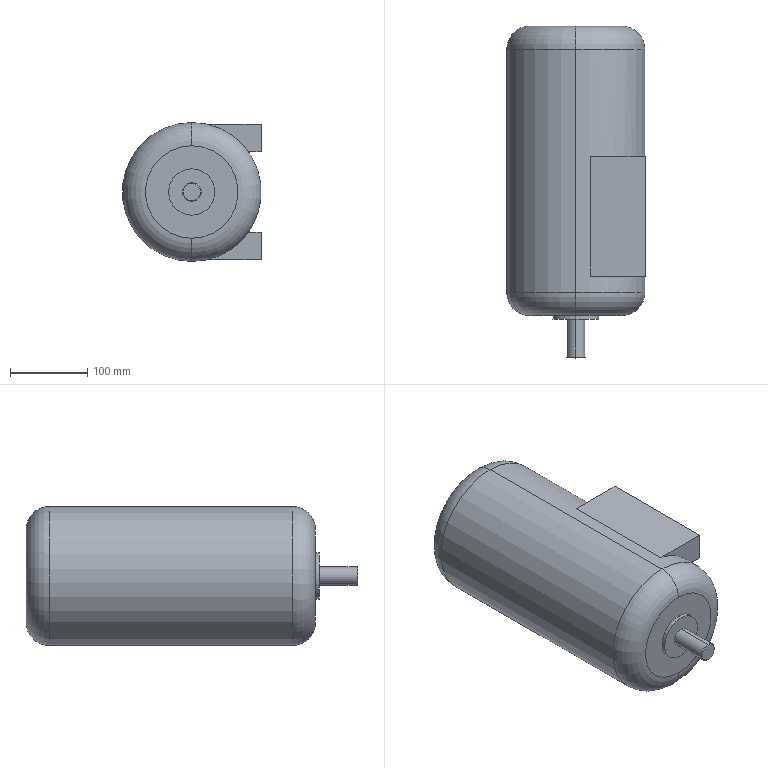Component | SolidWorks | YBBP-903-2-1.5Motor-1 | 1 solid | 26 faces | box 180 x 430 x 180 mm | volume 9782675 mm3 | plane 14 | cylinder 6 | torus 4 | cone 2 | commonest cylinder face diameters 60 x2 24 x2 180 x2 | material 45
build123d program:
from build123d import *

# Parameters (mm, degrees)
BOSS_EXTRUDE1_REACH      = 476.763
BOSS_EXTRUDE1_END_RADIUS = 90
SKETCH2_W                = 155
SKETCH2_H                = 36
FILLET1_R                = 30
CHAMFER1_SIZE            = 1


with BuildPart() as part:
    # Sketch1 → Revolve1 (revolve)
    with BuildSketch(Plane.XY, mode=Mode.PRIVATE) as revolve1_sk:
        Polygon((0, 0), (0, 12), (50, 12), (50, 30), (55, 30), (55, 90), (430, 90), (430, 0), align=None)
    revolve(revolve1_sk.sketch.rotate(Axis((0, 0, 0), (1, 0, 0)), 90), axis=Axis((0, 0, 0), (1, 0, 0)))

    # Boss-Extrude1: up to this cylinder (the profile starts outside it)
    boss_extrude1_end = Plane(origin=(183.5, 0, 0), z_dir=(-1, 0, 0)) * Cylinder(BOSS_EXTRUDE1_END_RADIUS, 1134.526, mode=Mode.PRIVATE)
    # Sketch2 → Boss-Extrude1 (add, up to the surface)
    with BuildSketch(Plane(origin=(0, -90, 0), x_dir=(1, 0, 0), z_dir=(0, 1, 0)), mode=Mode.PRIVATE) as boss_extrude1_sk1:
        with Locations((183.5, -70)):
            Rectangle(SKETCH2_W, SKETCH2_H)
    boss_extrude1_tool1 = extrude(boss_extrude1_sk1.sketch, amount=BOSS_EXTRUDE1_REACH, mode=Mode.PRIVATE) - boss_extrude1_end
    add(boss_extrude1_tool1.solids().sort_by_distance((183.5, -90, 70))[0])
    # Sketch2 → Boss-Extrude1 (add, up to the surface)
    with BuildSketch(Plane(origin=(0, -90, 0), x_dir=(1, 0, 0), z_dir=(0, 1, 0)), mode=Mode.PRIVATE) as boss_extrude1_sk2:
        with Locations((183.5, 70)):
            Rectangle(SKETCH2_W, SKETCH2_H)
    boss_extrude1_tool2 = extrude(boss_extrude1_sk2.sketch, amount=BOSS_EXTRUDE1_REACH, mode=Mode.PRIVATE) - boss_extrude1_end
    add(boss_extrude1_tool2.solids().sort_by_distance((183.5, -90, -70))[0])

    # Fillet1
    fillet1_edges = [part.edges().sort_by_distance(p)[0] for p in [
        (430, 0, -90),
        (55, 0, -90),
    ]]
    fillet(fillet1_edges, radius=FILLET1_R)

    # Chamfer1
    chamfer1_edges = [part.edges().sort_by_distance(p)[0] for p in [
        (0, 0, -12),
    ]]
    chamfer(chamfer1_edges, length=CHAMFER1_SIZE)


solid = part.part

# Placed as in the assembly
solid = solid.moved(Location((-371.359, -392.185, 1412), (0, 0, 90)))
STEP:
#1=COLOUR_RGB('',0.7922,0.8196,0.9333);
#2=FILL_AREA_STYLE_COLOUR('',#1);
#3=FILL_AREA_STYLE('',(#2));
#4=SURFACE_STYLE_FILL_AREA(#3);
#5=SURFACE_SIDE_STYLE('',(#4));
#6=SURFACE_STYLE_USAGE(.BOTH.,#5);
#7=PRESENTATION_STYLE_ASSIGNMENT((#6));
#8=CARTESIAN_POINT('',(-14.62,-15.44,56.024));
#9=VERTEX_POINT('',#8);
#10=CARTESIAN_POINT('',(-14.62,-15.44,55.157));
#11=VERTEX_POINT('',#10);
#12=CARTESIAN_POINT('',(-14.62,-15.44,55.591));
#13=DIRECTION('',(-0.,-1.,0.));
#14=DIRECTION('',(0.,0.,-1.));
#15=AXIS2_PLACEMENT_3D('',#12,#13,#14);
#16=CIRCLE('',#15,0.4331);
#17=EDGE_CURVE('',#9,#11,#16,.T.);
#18=ORIENTED_EDGE('',*,*,#17,.F.);
#19=CARTESIAN_POINT('',(-14.62,-15.401,56.063));
#20=VERTEX_POINT('',#19);
#21=CARTESIAN_POINT('',(-14.62,-15.44,56.024));
#22=DIRECTION('',(-0.,0.7071,0.7071));
#23=VECTOR('',#22,39.37);
#24=LINE('',#21,#23);
#25=EDGE_CURVE('',#9,#20,#24,.T.);
#26=ORIENTED_EDGE('',*,*,#25,.T.);
#27=CARTESIAN_POINT('',(-14.62,-15.401,55.118));
#28=VERTEX_POINT('',#27);
#29=CARTESIAN_POINT('',(-14.62,-15.401,55.591));
#30=DIRECTION('',(0.,1.,0.));
#31=DIRECTION('',(0.,0.,-1.));
#32=AXIS2_PLACEMENT_3D('',#29,#30,#31);
#33=CIRCLE('',#32,0.4724);
#34=EDGE_CURVE('',#28,#20,#33,.T.);
#35=ORIENTED_EDGE('',*,*,#34,.F.);
#36=CARTESIAN_POINT('',(-14.62,-15.44,55.157));
#37=DIRECTION('',(0.,0.7071,-0.7071));
#38=VECTOR('',#37,39.37);
#39=LINE('',#36,#38);
#40=EDGE_CURVE('',#11,#28,#39,.T.);
#41=ORIENTED_EDGE('',*,*,#40,.F.);
#42=EDGE_LOOP('',(#18,#26,#35,#41));
#43=FACE_OUTER_BOUND('',#42,.T.);
#44=CARTESIAN_POINT('',(-14.62,-15.44,55.591));
#45=DIRECTION('',(0.,1.,0.));
#46=DIRECTION('',(0.,0.,-1.));
#47=AXIS2_PLACEMENT_3D('',#44,#45,#46);
#48=CONICAL_SURFACE('',#47,0.4331,0.7854);
#49=ADVANCED_FACE('',(#43),#48,.T.);
#50=CARTESIAN_POINT('',(-14.62,1.489,53.228));
#51=VERTEX_POINT('',#50);
#52=CARTESIAN_POINT('',(-14.62,1.489,57.953));
#53=VERTEX_POINT('',#52);
#54=CARTESIAN_POINT('',(-14.62,1.489,55.591));
#55=DIRECTION('',(0.,1.,0.));
#56=DIRECTION('',(0.,0.,1.));
#57=AXIS2_PLACEMENT_3D('',#54,#55,#56);
#58=CIRCLE('',#57,2.362);
#59=EDGE_CURVE('',#51,#53,#58,.T.);
#60=ORIENTED_EDGE('',*,*,#59,.F.);
#61=CARTESIAN_POINT('',(-14.62,0.3077,52.047));
#62=VERTEX_POINT('',#61);
#63=CARTESIAN_POINT('',(-14.62,0.3077,53.228));
#64=DIRECTION('',(-1.,0.,0.));
#65=DIRECTION('',(0.,0.,1.));
#66=AXIS2_PLACEMENT_3D('',#63,#64,#65);
#67=CIRCLE('',#66,1.181);
#68=EDGE_CURVE('',#51,#62,#67,.T.);
#69=ORIENTED_EDGE('',*,*,#68,.T.);
#70=CARTESIAN_POINT('',(-14.62,0.3077,59.134));
#71=VERTEX_POINT('',#70);
#72=CARTESIAN_POINT('',(-14.62,0.3077,55.591));
#73=DIRECTION('',(-0.,-1.,0.));
#74=DIRECTION('',(0.,0.,1.));
#75=AXIS2_PLACEMENT_3D('',#72,#73,#74);
#76=CIRCLE('',#75,3.543);
#77=EDGE_CURVE('',#71,#62,#76,.T.);
#78=ORIENTED_EDGE('',*,*,#77,.F.);
#79=CARTESIAN_POINT('',(-14.62,0.3077,57.953));
#80=DIRECTION('',(1.,-0.,0.));
#81=DIRECTION('',(0.,1.,0.));
#82=AXIS2_PLACEMENT_3D('',#79,#80,#81);
#83=CIRCLE('',#82,1.181);
#84=EDGE_CURVE('',#53,#71,#83,.T.);
#85=ORIENTED_EDGE('',*,*,#84,.F.);
#86=EDGE_LOOP('',(#60,#69,#78,#85));
#87=FACE_OUTER_BOUND('',#86,.T.);
#88=CARTESIAN_POINT('',(-14.62,0.3077,55.591));
#89=DIRECTION('',(-0.,-1.,0.));
#90=DIRECTION('',(0.,0.,1.));
#91=AXIS2_PLACEMENT_3D('',#88,#89,#90);
#92=TOROIDAL_SURFACE('',#91,2.362,1.181);
#93=ADVANCED_FACE('',(#87),#92,.T.);
#94=CARTESIAN_POINT('',(-14.62,-13.275,57.953));
#95=VERTEX_POINT('',#94);
#96=CARTESIAN_POINT('',(-14.62,-13.275,53.228));
#97=VERTEX_POINT('',#96);
#98=CARTESIAN_POINT('',(-14.62,-13.275,55.591));
#99=DIRECTION('',(-0.,-1.,0.));
#100=DIRECTION('',(0.,0.,-1.));
#101=AXIS2_PLACEMENT_3D('',#98,#99,#100);
#102=CIRCLE('',#101,2.362);
#103=EDGE_CURVE('',#95,#97,#102,.T.);
#104=ORIENTED_EDGE('',*,*,#103,.F.);
#105=CARTESIAN_POINT('',(-14.62,-12.094,59.134));
#106=VERTEX_POINT('',#105);
#107=CARTESIAN_POINT('',(-14.62,-12.094,57.953));
#108=DIRECTION('',(-1.,0.,-0.));
#109=DIRECTION('',(0.,0.,1.));
#110=AXIS2_PLACEMENT_3D('',#107,#108,#109);
#111=CIRCLE('',#110,1.181);
#112=EDGE_CURVE('',#95,#106,#111,.T.);
#113=ORIENTED_EDGE('',*,*,#112,.T.);
#114=CARTESIAN_POINT('',(-14.62,-12.094,52.047));
#115=VERTEX_POINT('',#114);
#116=CARTESIAN_POINT('',(-14.62,-12.094,55.591));
#117=DIRECTION('',(0.,1.,0.));
#118=DIRECTION('',(0.,0.,-1.));
#119=AXIS2_PLACEMENT_3D('',#116,#117,#118);
#120=CIRCLE('',#119,3.543);
#121=EDGE_CURVE('',#115,#106,#120,.T.);
#122=ORIENTED_EDGE('',*,*,#121,.F.);
#123=CARTESIAN_POINT('',(-14.62,-12.094,53.228));
#124=DIRECTION('',(1.,-0.,0.));
#125=DIRECTION('',(0.,1.,0.));
#126=AXIS2_PLACEMENT_3D('',#123,#124,#125);
#127=CIRCLE('',#126,1.181);
#128=EDGE_CURVE('',#97,#115,#127,.T.);
#129=ORIENTED_EDGE('',*,*,#128,.F.);
#130=EDGE_LOOP('',(#104,#113,#122,#129));
#131=FACE_OUTER_BOUND('',#130,.T.);
#132=CARTESIAN_POINT('',(-14.62,-12.094,55.591));
#133=DIRECTION('',(0.,1.,0.));
#134=DIRECTION('',(0.,0.,-1.));
#135=AXIS2_PLACEMENT_3D('',#132,#133,#134);
#136=TOROIDAL_SURFACE('',#135,2.362,1.181);
#137=ADVANCED_FACE('',(#131),#136,.T.);
#138=CARTESIAN_POINT('',(-14.62,-13.275,56.772));
#139=VERTEX_POINT('',#138);
#140=CARTESIAN_POINT('',(-14.62,-13.275,54.409));
#141=VERTEX_POINT('',#140);
#142=CARTESIAN_POINT('',(-14.62,-13.275,55.591));
#143=DIRECTION('',(-0.,-1.,0.));
#144=DIRECTION('',(0.,0.,1.));
#145=AXIS2_PLACEMENT_3D('',#142,#143,#144);
#146=CIRCLE('',#145,1.181);
#147=EDGE_CURVE('',#139,#141,#146,.T.);
#148=ORIENTED_EDGE('',*,*,#147,.T.);
#149=CARTESIAN_POINT('',(-14.62,-13.472,54.409));
#150=VERTEX_POINT('',#149);
#151=CARTESIAN_POINT('',(-14.62,-15.44,54.409));
#152=DIRECTION('',(-0.,-1.,0.));
#153=VECTOR('',#152,39.37);
#154=LINE('',#151,#153);
#155=EDGE_CURVE('',#141,#150,#154,.T.);
#156=ORIENTED_EDGE('',*,*,#155,.T.);
#157=CARTESIAN_POINT('',(-14.62,-13.472,56.772));
#158=VERTEX_POINT('',#157);
#159=CARTESIAN_POINT('',(-14.62,-13.472,55.591));
#160=DIRECTION('',(-0.,-1.,0.));
#161=DIRECTION('',(0.,0.,1.));
#162=AXIS2_PLACEMENT_3D('',#159,#160,#161);
#163=CIRCLE('',#162,1.181);
#164=EDGE_CURVE('',#158,#150,#163,.T.);
#165=ORIENTED_EDGE('',*,*,#164,.F.);
#166=CARTESIAN_POINT('',(-14.62,-15.44,56.772));
#167=DIRECTION('',(-0.,-1.,0.));
#168=VECTOR('',#167,39.37);
#169=LINE('',#166,#168);
#170=EDGE_CURVE('',#139,#158,#169,.T.);
#171=ORIENTED_EDGE('',*,*,#170,.F.);
#172=EDGE_LOOP('',(#148,#156,#165,#171));
#173=FACE_OUTER_BOUND('',#172,.T.);
#174=CARTESIAN_POINT('',(-14.62,-15.44,55.591));
#175=DIRECTION('',(-0.,-1.,0.));
#176=DIRECTION('',(0.,0.,1.));
#177=AXIS2_PLACEMENT_3D('',#174,#175,#176);
#178=CYLINDRICAL_SURFACE('',#177,1.181);
#179=ADVANCED_FACE('',(#173),#178,.T.);
#180=CARTESIAN_POINT('',(-14.62,-13.472,56.063));
#181=VERTEX_POINT('',#180);
#182=CARTESIAN_POINT('',(-14.62,-13.472,55.118));
#183=VERTEX_POINT('',#182);
#184=CARTESIAN_POINT('',(-14.62,-13.472,55.591));
#185=DIRECTION('',(-0.,-1.,0.));
#186=DIRECTION('',(0.,0.,1.));
#187=AXIS2_PLACEMENT_3D('',#184,#185,#186);
#188=CIRCLE('',#187,0.4724);
#189=EDGE_CURVE('',#181,#183,#188,.T.);
#190=ORIENTED_EDGE('',*,*,#189,.T.);
#191=CARTESIAN_POINT('',(-14.62,-15.44,55.118));
#192=DIRECTION('',(-0.,-1.,0.));
#193=VECTOR('',#192,39.37);
#194=LINE('',#191,#193);
#195=EDGE_CURVE('',#183,#28,#194,.T.);
#196=ORIENTED_EDGE('',*,*,#195,.T.);
#197=ORIENTED_EDGE('',*,*,#34,.T.);
#198=CARTESIAN_POINT('',(-14.62,-15.44,56.063));
#199=DIRECTION('',(-0.,-1.,0.));
#200=VECTOR('',#199,39.37);
#201=LINE('',#198,#200);
#202=EDGE_CURVE('',#181,#20,#201,.T.);
#203=ORIENTED_EDGE('',*,*,#202,.F.);
#204=EDGE_LOOP('',(#190,#196,#197,#203));
#205=FACE_OUTER_BOUND('',#204,.T.);
#206=CARTESIAN_POINT('',(-14.62,-15.44,55.591));
#207=DIRECTION('',(-0.,-1.,0.));
#208=DIRECTION('',(0.,0.,1.));
#209=AXIS2_PLACEMENT_3D('',#206,#207,#208);
#210=CYLINDRICAL_SURFACE('',#209,0.4724);
#211=ADVANCED_FACE('',(#205),#210,.T.);
#212=ORIENTED_EDGE('',*,*,#77,.T.);
#213=CARTESIAN_POINT('',(-14.62,-15.44,52.047));
#214=DIRECTION('',(-0.,-1.,0.));
#215=VECTOR('',#214,39.37);
#216=LINE('',#213,#215);
#217=EDGE_CURVE('',#62,#115,#216,.T.);
#218=ORIENTED_EDGE('',*,*,#217,.T.);
#219=ORIENTED_EDGE('',*,*,#121,.T.);
#220=CARTESIAN_POINT('',(-14.62,-15.44,59.134));
#221=DIRECTION('',(-0.,-1.,0.));
#222=VECTOR('',#221,39.37);
#223=LINE('',#220,#222);
#224=EDGE_CURVE('',#71,#106,#223,.T.);
#225=ORIENTED_EDGE('',*,*,#224,.F.);
#226=EDGE_LOOP('',(#212,#218,#219,#225));
#227=FACE_OUTER_BOUND('',#226,.T.);
#228=CARTESIAN_POINT('',(-14.62,-15.44,55.591));
#229=DIRECTION('',(-0.,-1.,0.));
#230=DIRECTION('',(0.,0.,1.));
#231=AXIS2_PLACEMENT_3D('',#228,#229,#230);
#232=CYLINDRICAL_SURFACE('',#231,3.543);
#233=ADVANCED_FACE('',(#227),#232,.T.);
#234=ORIENTED_EDGE('',*,*,#217,.F.);
#235=CARTESIAN_POINT('',(-14.62,0.3077,55.591));
#236=DIRECTION('',(-0.,-1.,0.));
#237=DIRECTION('',(0.,0.,1.));
#238=AXIS2_PLACEMENT_3D('',#235,#236,#237);
#239=CIRCLE('',#238,3.543);
#240=EDGE_CURVE('',#62,#71,#239,.T.);
#241=ORIENTED_EDGE('',*,*,#240,.T.);
#242=ORIENTED_EDGE('',*,*,#224,.T.);
#243=CARTESIAN_POINT('',(-14.62,-12.094,55.591));
#244=DIRECTION('',(0.,1.,0.));
#245=DIRECTION('',(0.,0.,-1.));
#246=AXIS2_PLACEMENT_3D('',#243,#244,#245);
#247=CIRCLE('',#246,3.543);
#248=EDGE_CURVE('',#106,#115,#247,.T.);
#249=ORIENTED_EDGE('',*,*,#248,.T.);
#250=EDGE_LOOP('',(#234,#241,#242,#249));
#251=FACE_OUTER_BOUND('',#250,.T.);
#252=CARTESIAN_POINT('',(-13.878,-11.267,59.055));
#253=VERTEX_POINT('',#252);
#254=CARTESIAN_POINT('',(-13.878,-5.165,59.055));
#255=VERTEX_POINT('',#254);
#256=CARTESIAN_POINT('',(-13.878,-15.44,59.055));
#257=DIRECTION('',(0.,1.,0.));
#258=VECTOR('',#257,39.37);
#259=LINE('',#256,#258);
#260=EDGE_CURVE('',#253,#255,#259,.T.);
#261=ORIENTED_EDGE('',*,*,#260,.T.);
#262=CARTESIAN_POINT('',(-11.728,-5.165,57.638));
#263=VERTEX_POINT('',#262);
#264=CARTESIAN_POINT('',(-14.62,-5.165,55.591));
#265=DIRECTION('',(0.,1.,0.));
#266=DIRECTION('',(0.,0.,1.));
#267=AXIS2_PLACEMENT_3D('',#264,#265,#266);
#268=CIRCLE('',#267,3.543);
#269=EDGE_CURVE('',#255,#263,#268,.T.);
#270=ORIENTED_EDGE('',*,*,#269,.T.);
#271=CARTESIAN_POINT('',(-11.728,-11.267,57.638));
#272=VERTEX_POINT('',#271);
#273=CARTESIAN_POINT('',(-11.728,-15.44,57.638));
#274=DIRECTION('',(-0.,-1.,0.));
#275=VECTOR('',#274,39.37);
#276=LINE('',#273,#275);
#277=EDGE_CURVE('',#263,#272,#276,.T.);
#278=ORIENTED_EDGE('',*,*,#277,.T.);
#279=CARTESIAN_POINT('',(-14.62,-11.267,55.591));
#280=DIRECTION('',(-0.,-1.,0.));
#281=DIRECTION('',(0.,-0.,-1.));
#282=AXIS2_PLACEMENT_3D('',#279,#280,#281);
#283=CIRCLE('',#282,3.543);
#284=EDGE_CURVE('',#272,#253,#283,.T.);
#285=ORIENTED_EDGE('',*,*,#284,.T.);
#286=EDGE_LOOP('',(#261,#270,#278,#285));
#287=FACE_BOUND('',#286,.T.);
#288=CARTESIAN_POINT('',(-11.728,-11.267,53.543));
#289=VERTEX_POINT('',#288);
#290=CARTESIAN_POINT('',(-11.728,-5.165,53.543));
#291=VERTEX_POINT('',#290);
#292=CARTESIAN_POINT('',(-11.728,-15.44,53.543));
#293=DIRECTION('',(0.,1.,0.));
#294=VECTOR('',#293,39.37);
#295=LINE('',#292,#294);
#296=EDGE_CURVE('',#289,#291,#295,.T.);
#297=ORIENTED_EDGE('',*,*,#296,.T.);
#298=CARTESIAN_POINT('',(-13.878,-5.165,52.126));
#299=VERTEX_POINT('',#298);
#300=CARTESIAN_POINT('',(-14.62,-5.165,55.591));
#301=DIRECTION('',(0.,1.,0.));
#302=DIRECTION('',(0.,0.,1.));
#303=AXIS2_PLACEMENT_3D('',#300,#301,#302);
#304=CIRCLE('',#303,3.543);
#305=EDGE_CURVE('',#291,#299,#304,.T.);
#306=ORIENTED_EDGE('',*,*,#305,.T.);
#307=CARTESIAN_POINT('',(-13.878,-11.267,52.126));
#308=VERTEX_POINT('',#307);
#309=CARTESIAN_POINT('',(-13.878,-15.44,52.126));
#310=DIRECTION('',(-0.,-1.,0.));
#311=VECTOR('',#310,39.37);
#312=LINE('',#309,#311);
#313=EDGE_CURVE('',#299,#308,#312,.T.);
#314=ORIENTED_EDGE('',*,*,#313,.T.);
#315=CARTESIAN_POINT('',(-14.62,-11.267,55.591));
#316=DIRECTION('',(-0.,-1.,0.));
#317=DIRECTION('',(0.,0.,-1.));
#318=AXIS2_PLACEMENT_3D('',#315,#316,#317);
#319=CIRCLE('',#318,3.543);
#320=EDGE_CURVE('',#308,#289,#319,.T.);
#321=ORIENTED_EDGE('',*,*,#320,.T.);
#322=EDGE_LOOP('',(#297,#306,#314,#321));
#323=FACE_BOUND('',#322,.T.);
#324=CARTESIAN_POINT('',(-14.62,-15.44,55.591));
#325=DIRECTION('',(-0.,-1.,0.));
#326=DIRECTION('',(0.,0.,1.));
#327=AXIS2_PLACEMENT_3D('',#324,#325,#326);
#328=CYLINDRICAL_SURFACE('',#327,3.543);
#329=ADVANCED_FACE('',(#251,#287,#323),#328,.T.);
#330=CARTESIAN_POINT('',(-14.62,-15.44,55.591));
#331=DIRECTION('',(-0.,-1.,0.));
#332=DIRECTION('',(0.,0.,-1.));
#333=AXIS2_PLACEMENT_3D('',#330,#331,#332);
#334=CIRCLE('',#333,0.4331);
#335=EDGE_CURVE('',#11,#9,#334,.T.);
#336=ORIENTED_EDGE('',*,*,#335,.T.);
#337=ORIENTED_EDGE('',*,*,#17,.T.);
#338=EDGE_LOOP('',(#336,#337));
#339=FACE_OUTER_BOUND('',#338,.T.);
#340=CARTESIAN_POINT('',(-14.62,-15.44,55.591));
#341=DIRECTION('',(0.,1.,0.));
#342=DIRECTION('',(0.,0.,-1.));
#343=AXIS2_PLACEMENT_3D('',#340,#341,#342);
#344=PLANE('',#343);
#345=ADVANCED_FACE('',(#339),#344,.F.);
#346=ORIENTED_EDGE('',*,*,#195,.F.);
#347=CARTESIAN_POINT('',(-14.62,-13.472,55.591));
#348=DIRECTION('',(-0.,-1.,0.));
#349=DIRECTION('',(0.,0.,1.));
#350=AXIS2_PLACEMENT_3D('',#347,#348,#349);
#351=CIRCLE('',#350,0.4724);
#352=EDGE_CURVE('',#183,#181,#351,.T.);
#353=ORIENTED_EDGE('',*,*,#352,.T.);
#354=ORIENTED_EDGE('',*,*,#202,.T.);
#355=CARTESIAN_POINT('',(-14.62,-15.401,55.591));
#356=DIRECTION('',(0.,1.,0.));
#357=DIRECTION('',(0.,0.,-1.));
#358=AXIS2_PLACEMENT_3D('',#355,#356,#357);
#359=CIRCLE('',#358,0.4724);
#360=EDGE_CURVE('',#20,#28,#359,.T.);
#361=ORIENTED_EDGE('',*,*,#360,.T.);
#362=EDGE_LOOP('',(#346,#353,#354,#361));
#363=FACE_OUTER_BOUND('',#362,.T.);
#364=CARTESIAN_POINT('',(-14.62,-15.44,55.591));
#365=DIRECTION('',(-0.,-1.,0.));
#366=DIRECTION('',(0.,0.,1.));
#367=AXIS2_PLACEMENT_3D('',#364,#365,#366);
#368=CYLINDRICAL_SURFACE('',#367,0.4724);
#369=ADVANCED_FACE('',(#363),#368,.T.);
#370=ORIENTED_EDGE('',*,*,#189,.F.);
#371=ORIENTED_EDGE('',*,*,#352,.F.);
#372=EDGE_LOOP('',(#370,#371));
#373=FACE_BOUND('',#372,.T.);
#374=ORIENTED_EDGE('',*,*,#164,.T.);
#375=CARTESIAN_POINT('',(-14.62,-13.472,55.591));
#376=DIRECTION('',(-0.,-1.,0.));
#377=DIRECTION('',(0.,0.,1.));
#378=AXIS2_PLACEMENT_3D('',#375,#376,#377);
#379=CIRCLE('',#378,1.181);
#380=EDGE_CURVE('',#150,#158,#379,.T.);
#381=ORIENTED_EDGE('',*,*,#380,.T.);
#382=EDGE_LOOP('',(#374,#381));
#383=FACE_OUTER_BOUND('',#382,.T.);
#384=CARTESIAN_POINT('',(-15.093,-13.472,55.591));
#385=DIRECTION('',(0.,1.,0.));
#386=DIRECTION('',(0.,0.,-1.));
#387=AXIS2_PLACEMENT_3D('',#384,#385,#386);
#388=PLANE('',#387);
#389=ADVANCED_FACE('',(#373,#383),#388,.F.);
#390=ORIENTED_EDGE('',*,*,#155,.F.);
#391=CARTESIAN_POINT('',(-14.62,-13.275,55.591));
#392=DIRECTION('',(-0.,-1.,0.));
#393=DIRECTION('',(0.,0.,1.));
#394=AXIS2_PLACEMENT_3D('',#391,#392,#393);
#395=CIRCLE('',#394,1.181);
#396=EDGE_CURVE('',#141,#139,#395,.T.);
#397=ORIENTED_EDGE('',*,*,#396,.T.);
#398=ORIENTED_EDGE('',*,*,#170,.T.);
#399=ORIENTED_EDGE('',*,*,#380,.F.);
#400=EDGE_LOOP('',(#390,#397,#398,#399));
#401=FACE_OUTER_BOUND('',#400,.T.);
#402=CARTESIAN_POINT('',(-14.62,-15.44,55.591));
#403=DIRECTION('',(-0.,-1.,0.));
#404=DIRECTION('',(0.,0.,1.));
#405=AXIS2_PLACEMENT_3D('',#402,#403,#404);
#406=CYLINDRICAL_SURFACE('',#405,1.181);
#407=ADVANCED_FACE('',(#401),#406,.T.);
#408=CARTESIAN_POINT('',(-14.62,-13.275,55.591));
#409=DIRECTION('',(-0.,-1.,0.));
#410=DIRECTION('',(0.,0.,-1.));
#411=AXIS2_PLACEMENT_3D('',#408,#409,#410);
#412=CIRCLE('',#411,2.362);
#413=EDGE_CURVE('',#97,#95,#412,.T.);
#414=ORIENTED_EDGE('',*,*,#413,.T.);
#415=ORIENTED_EDGE('',*,*,#103,.T.);
#416=EDGE_LOOP('',(#414,#415));
#417=FACE_OUTER_BOUND('',#416,.T.);
#418=ORIENTED_EDGE('',*,*,#147,.F.);
#419=ORIENTED_EDGE('',*,*,#396,.F.);
#420=EDGE_LOOP('',(#418,#419));
#421=FACE_BOUND('',#420,.T.);
#422=CARTESIAN_POINT('',(-15.802,-13.275,55.591));
#423=DIRECTION('',(0.,1.,0.));
#424=DIRECTION('',(0.,0.,-1.));
#425=AXIS2_PLACEMENT_3D('',#422,#423,#424);
#426=PLANE('',#425);
#427=ADVANCED_FACE('',(#417,#421),#426,.F.);
#428=CARTESIAN_POINT('',(-14.62,1.489,55.591));
#429=DIRECTION('',(0.,1.,0.));
#430=DIRECTION('',(0.,0.,1.));
#431=AXIS2_PLACEMENT_3D('',#428,#429,#430);
#432=CIRCLE('',#431,2.362);
#433=EDGE_CURVE('',#53,#51,#432,.T.);
#434=ORIENTED_EDGE('',*,*,#433,.T.);
#435=ORIENTED_EDGE('',*,*,#59,.T.);
#436=EDGE_LOOP('',(#434,#435));
#437=FACE_OUTER_BOUND('',#436,.T.);
#438=CARTESIAN_POINT('',(-18.164,1.489,55.591));
#439=DIRECTION('',(-0.,-1.,0.));
#440=DIRECTION('',(0.,0.,1.));
#441=AXIS2_PLACEMENT_3D('',#438,#439,#440);
#442=PLANE('',#441);
#443=ADVANCED_FACE('',(#437),#442,.F.);
#444=ORIENTED_EDGE('',*,*,#277,.F.);
#445=CARTESIAN_POINT('',(-11.077,-5.165,57.638));
#446=VERTEX_POINT('',#445);
#447=CARTESIAN_POINT('',(-19699.66,-5.165,57.638));
#448=DIRECTION('',(1.,-0.,0.));
#449=VECTOR('',#448,39.37);
#450=LINE('',#447,#449);
#451=EDGE_CURVE('',#263,#446,#450,.T.);
#452=ORIENTED_EDGE('',*,*,#451,.T.);
#453=CARTESIAN_POINT('',(-11.077,-11.267,57.638));
#454=VERTEX_POINT('',#453);
#455=CARTESIAN_POINT('',(-11.077,-5.165,57.638));
#456=DIRECTION('',(-0.,-1.,0.));
#457=VECTOR('',#456,39.37);
#458=LINE('',#455,#457);
#459=EDGE_CURVE('',#446,#454,#458,.T.);
#460=ORIENTED_EDGE('',*,*,#459,.T.);
#461=CARTESIAN_POINT('',(-19699.66,-11.267,57.638));
#462=DIRECTION('',(1.,-0.,0.));
#463=VECTOR('',#462,39.37);
#464=LINE('',#461,#463);
#465=EDGE_CURVE('',#272,#454,#464,.T.);
#466=ORIENTED_EDGE('',*,*,#465,.F.);
#467=EDGE_LOOP('',(#444,#452,#460,#466));
#468=FACE_OUTER_BOUND('',#467,.T.);
#469=CARTESIAN_POINT('',(-19699.66,-5.165,57.638));
#470=DIRECTION('',(0.,0.,1.));
#471=DIRECTION('',(0.,1.,-0.));
#472=AXIS2_PLACEMENT_3D('',#469,#470,#471);
#473=PLANE('',#472);
#474=ADVANCED_FACE('',(#468),#473,.F.);
#475=ORIENTED_EDGE('',*,*,#269,.F.);
#476=CARTESIAN_POINT('',(-11.077,-5.165,59.055));
#477=VERTEX_POINT('',#476);
#478=CARTESIAN_POINT('',(-19699.66,-5.165,59.055));
#479=DIRECTION('',(1.,-0.,0.));
#480=VECTOR('',#479,39.37);
#481=LINE('',#478,#480);
#482=EDGE_CURVE('',#255,#477,#481,.T.);
#483=ORIENTED_EDGE('',*,*,#482,.T.);
#484=CARTESIAN_POINT('',(-11.077,-5.165,57.638));
#485=DIRECTION('',(0.,0.,-1.));
#486=VECTOR('',#485,39.37);
#487=LINE('',#484,#486);
#488=EDGE_CURVE('',#477,#446,#487,.T.);
#489=ORIENTED_EDGE('',*,*,#488,.T.);
#490=ORIENTED_EDGE('',*,*,#451,.F.);
#491=EDGE_LOOP('',(#475,#483,#489,#490));
#492=FACE_OUTER_BOUND('',#491,.T.);
#493=CARTESIAN_POINT('',(-19699.66,-5.165,57.638));
#494=DIRECTION('',(-0.,-1.,0.));
#495=DIRECTION('',(0.,0.,1.));
#496=AXIS2_PLACEMENT_3D('',#493,#494,#495);
#497=PLANE('',#496);
#498=ADVANCED_FACE('',(#492),#497,.F.);
#499=CARTESIAN_POINT('',(-11.077,-11.267,59.055));
#500=VERTEX_POINT('',#499);
#501=CARTESIAN_POINT('',(-11.077,-11.267,57.638));
#502=DIRECTION('',(0.,0.,1.));
#503=VECTOR('',#502,39.37);
#504=LINE('',#501,#503);
#505=EDGE_CURVE('',#454,#500,#504,.T.);
#506=ORIENTED_EDGE('',*,*,#505,.F.);
#507=ORIENTED_EDGE('',*,*,#459,.F.);
#508=ORIENTED_EDGE('',*,*,#488,.F.);
#509=CARTESIAN_POINT('',(-11.077,-5.165,59.055));
#510=DIRECTION('',(0.,1.,0.));
#511=VECTOR('',#510,39.37);
#512=LINE('',#509,#511);
#513=EDGE_CURVE('',#500,#477,#512,.T.);
#514=ORIENTED_EDGE('',*,*,#513,.F.);
#515=EDGE_LOOP('',(#506,#507,#508,#514));
#516=FACE_OUTER_BOUND('',#515,.T.);
#517=CARTESIAN_POINT('',(-11.077,-15.44,55.591));
#518=DIRECTION('',(1.,-0.,0.));
#519=DIRECTION('',(0.,0.,-1.));
#520=AXIS2_PLACEMENT_3D('',#517,#518,#519);
#521=PLANE('',#520);
#522=ADVANCED_FACE('',(#516),#521,.T.);
#523=ORIENTED_EDGE('',*,*,#284,.F.);
#524=ORIENTED_EDGE('',*,*,#465,.T.);
#525=ORIENTED_EDGE('',*,*,#505,.T.);
#526=CARTESIAN_POINT('',(-19699.66,-11.267,59.055));
#527=DIRECTION('',(1.,-0.,0.));
#528=VECTOR('',#527,39.37);
#529=LINE('',#526,#528);
#530=EDGE_CURVE('',#253,#500,#529,.T.);
#531=ORIENTED_EDGE('',*,*,#530,.F.);
#532=EDGE_LOOP('',(#523,#524,#525,#531));
#533=FACE_OUTER_BOUND('',#532,.T.);
#534=CARTESIAN_POINT('',(-19699.66,-11.267,57.638));
#535=DIRECTION('',(0.,1.,-0.));
#536=DIRECTION('',(-0.,-0.,-1.));
#537=AXIS2_PLACEMENT_3D('',#534,#535,#536);
#538=PLANE('',#537);
#539=ADVANCED_FACE('',(#533),#538,.F.);
#540=ORIENTED_EDGE('',*,*,#260,.F.);
#541=ORIENTED_EDGE('',*,*,#530,.T.);
#542=ORIENTED_EDGE('',*,*,#513,.T.);
#543=ORIENTED_EDGE('',*,*,#482,.F.);
#544=EDGE_LOOP('',(#540,#541,#542,#543));
#545=FACE_OUTER_BOUND('',#544,.T.);
#546=CARTESIAN_POINT('',(-19699.66,-5.165,59.055));
#547=DIRECTION('',(0.,0.,-1.));
#548=DIRECTION('',(-0.,-1.,0.));
#549=AXIS2_PLACEMENT_3D('',#546,#547,#548);
#550=PLANE('',#549);
#551=ADVANCED_FACE('',(#545),#550,.F.);
#552=ORIENTED_EDGE('',*,*,#313,.F.);
#553=CARTESIAN_POINT('',(-11.077,-5.165,52.126));
#554=VERTEX_POINT('',#553);
#555=CARTESIAN_POINT('',(-19699.66,-5.165,52.126));
#556=DIRECTION('',(1.,-0.,0.));
#557=VECTOR('',#556,39.37);
#558=LINE('',#555,#557);
#559=EDGE_CURVE('',#299,#554,#558,.T.);
#560=ORIENTED_EDGE('',*,*,#559,.T.);
#561=CARTESIAN_POINT('',(-11.077,-11.267,52.126));
#562=VERTEX_POINT('',#561);
#563=CARTESIAN_POINT('',(-11.077,-5.165,52.126));
#564=DIRECTION('',(-0.,-1.,0.));
#565=VECTOR('',#564,39.37);
#566=LINE('',#563,#565);
#567=EDGE_CURVE('',#554,#562,#566,.T.);
#568=ORIENTED_EDGE('',*,*,#567,.T.);
#569=CARTESIAN_POINT('',(-19699.66,-11.267,52.126));
#570=DIRECTION('',(1.,-0.,0.));
#571=VECTOR('',#570,39.37);
#572=LINE('',#569,#571);
#573=EDGE_CURVE('',#308,#562,#572,.T.);
#574=ORIENTED_EDGE('',*,*,#573,.F.);
#575=EDGE_LOOP('',(#552,#560,#568,#574));
#576=FACE_OUTER_BOUND('',#575,.T.);
#577=CARTESIAN_POINT('',(-19699.66,-5.165,52.126));
#578=DIRECTION('',(0.,0.,1.));
#579=DIRECTION('',(0.,1.,0.));
#580=AXIS2_PLACEMENT_3D('',#577,#578,#579);
#581=PLANE('',#580);
#582=ADVANCED_FACE('',(#576),#581,.F.);
#583=ORIENTED_EDGE('',*,*,#305,.F.);
#584=CARTESIAN_POINT('',(-11.077,-5.165,53.543));
#585=VERTEX_POINT('',#584);
#586=CARTESIAN_POINT('',(-19699.66,-5.165,53.543));
#587=DIRECTION('',(1.,-0.,0.));
#588=VECTOR('',#587,39.37);
#589=LINE('',#586,#588);
#590=EDGE_CURVE('',#291,#585,#589,.T.);
#591=ORIENTED_EDGE('',*,*,#590,.T.);
#592=CARTESIAN_POINT('',(-11.077,-5.165,52.126));
#593=DIRECTION('',(0.,0.,-1.));
#594=VECTOR('',#593,39.37);
#595=LINE('',#592,#594);
#596=EDGE_CURVE('',#585,#554,#595,.T.);
#597=ORIENTED_EDGE('',*,*,#596,.T.);
#598=ORIENTED_EDGE('',*,*,#559,.F.);
#599=EDGE_LOOP('',(#583,#591,#597,#598));
#600=FACE_OUTER_BOUND('',#599,.T.);
#601=CARTESIAN_POINT('',(-19699.66,-5.165,52.126));
#602=DIRECTION('',(-0.,-1.,0.));
#603=DIRECTION('',(0.,0.,1.));
#604=AXIS2_PLACEMENT_3D('',#601,#602,#603);
#605=PLANE('',#604);
#606=ADVANCED_FACE('',(#600),#605,.F.);
#607=CARTESIAN_POINT('',(-11.077,-11.267,53.543));
#608=VERTEX_POINT('',#607);
#609=CARTESIAN_POINT('',(-11.077,-11.267,52.126));
#610=DIRECTION('',(0.,0.,1.));
#611=VECTOR('',#610,39.37);
#612=LINE('',#609,#611);
#613=EDGE_CURVE('',#562,#608,#612,.T.);
#614=ORIENTED_EDGE('',*,*,#613,.F.);
#615=ORIENTED_EDGE('',*,*,#567,.F.);
#616=ORIENTED_EDGE('',*,*,#596,.F.);
#617=CARTESIAN_POINT('',(-11.077,-5.165,53.543));
#618=DIRECTION('',(0.,1.,0.));
#619=VECTOR('',#618,39.37);
#620=LINE('',#617,#619);
#621=EDGE_CURVE('',#608,#585,#620,.T.);
#622=ORIENTED_EDGE('',*,*,#621,.F.);
#623=EDGE_LOOP('',(#614,#615,#616,#622));
#624=FACE_OUTER_BOUND('',#623,.T.);
#625=CARTESIAN_POINT('',(-11.077,-15.44,55.591));
#626=DIRECTION('',(1.,-0.,0.));
#627=DIRECTION('',(0.,0.,-1.));
#628=AXIS2_PLACEMENT_3D('',#625,#626,#627);
#629=PLANE('',#628);
#630=ADVANCED_FACE('',(#624),#629,.T.);
#631=ORIENTED_EDGE('',*,*,#320,.F.);
#632=ORIENTED_EDGE('',*,*,#573,.T.);
#633=ORIENTED_EDGE('',*,*,#613,.T.);
#634=CARTESIAN_POINT('',(-19699.66,-11.267,53.543));
#635=DIRECTION('',(1.,-0.,0.));
#636=VECTOR('',#635,39.37);
#637=LINE('',#634,#636);
#638=EDGE_CURVE('',#289,#608,#637,.T.);
#639=ORIENTED_EDGE('',*,*,#638,.F.);
#640=EDGE_LOOP('',(#631,#632,#633,#639));
#641=FACE_OUTER_BOUND('',#640,.T.);
#642=CARTESIAN_POINT('',(-19699.66,-11.267,52.126));
#643=DIRECTION('',(0.,1.,0.));
#644=DIRECTION('',(0.,0.,-1.));
#645=AXIS2_PLACEMENT_3D('',#642,#643,#644);
#646=PLANE('',#645);
#647=ADVANCED_FACE('',(#641),#646,.F.);
#648=ORIENTED_EDGE('',*,*,#296,.F.);
#649=ORIENTED_EDGE('',*,*,#638,.T.);
#650=ORIENTED_EDGE('',*,*,#621,.T.);
#651=ORIENTED_EDGE('',*,*,#590,.F.);
#652=EDGE_LOOP('',(#648,#649,#650,#651));
#653=FACE_OUTER_BOUND('',#652,.T.);
#654=CARTESIAN_POINT('',(-19699.66,-5.165,53.543));
#655=DIRECTION('',(0.,0.,-1.));
#656=DIRECTION('',(-0.,-1.,0.));
#657=AXIS2_PLACEMENT_3D('',#654,#655,#656);
#658=PLANE('',#657);
#659=ADVANCED_FACE('',(#653),#658,.F.);
#660=ORIENTED_EDGE('',*,*,#112,.F.);
#661=ORIENTED_EDGE('',*,*,#413,.F.);
#662=ORIENTED_EDGE('',*,*,#128,.T.);
#663=ORIENTED_EDGE('',*,*,#248,.F.);
#664=EDGE_LOOP('',(#660,#661,#662,#663));
#665=FACE_OUTER_BOUND('',#664,.T.);
#666=CARTESIAN_POINT('',(-14.62,-12.094,55.591));
#667=DIRECTION('',(0.,1.,0.));
#668=DIRECTION('',(0.,0.,-1.));
#669=AXIS2_PLACEMENT_3D('',#666,#667,#668);
#670=TOROIDAL_SURFACE('',#669,2.362,1.181);
#671=ADVANCED_FACE('',(#665),#670,.T.);
#672=ORIENTED_EDGE('',*,*,#68,.F.);
#673=ORIENTED_EDGE('',*,*,#433,.F.);
#674=ORIENTED_EDGE('',*,*,#84,.T.);
#675=ORIENTED_EDGE('',*,*,#240,.F.);
#676=EDGE_LOOP('',(#672,#673,#674,#675));
#677=FACE_OUTER_BOUND('',#676,.T.);
#678=CARTESIAN_POINT('',(-14.62,0.3077,55.591));
#679=DIRECTION('',(-0.,-1.,0.));
#680=DIRECTION('',(0.,0.,1.));
#681=AXIS2_PLACEMENT_3D('',#678,#679,#680);
#682=TOROIDAL_SURFACE('',#681,2.362,1.181);
#683=ADVANCED_FACE('',(#677),#682,.T.);
#684=ORIENTED_EDGE('',*,*,#25,.F.);
#685=ORIENTED_EDGE('',*,*,#335,.F.);
#686=ORIENTED_EDGE('',*,*,#40,.T.);
#687=ORIENTED_EDGE('',*,*,#360,.F.);
#688=EDGE_LOOP('',(#684,#685,#686,#687));
#689=FACE_OUTER_BOUND('',#688,.T.);
#690=CARTESIAN_POINT('',(-14.62,-15.44,55.591));
#691=DIRECTION('',(0.,1.,0.));
#692=DIRECTION('',(0.,0.,-1.));
#693=AXIS2_PLACEMENT_3D('',#690,#691,#692);
#694=CONICAL_SURFACE('',#693,0.4331,0.7854);
#695=ADVANCED_FACE('',(#689),#694,.T.);
#696=CLOSED_SHELL('',(#49,#93,#137,#179,#211,#233,#329,#345,#369,#389,#407,#427,#443,#474,#498,#522,#539,#551,#582,#606,#630,#647,#659,#671,#683,#695));
#697=MANIFOLD_SOLID_BREP('',#696);
#698=STYLED_ITEM('',(#7),#697);
#699=PRESENTATION_LAYER_ASSIGNMENT('','',(#698));
#700=CARTESIAN_POINT('',(0.,0.,0.));
#701=DIRECTION('',(0.,0.,1.));
#702=DIRECTION('',(1.,0.,0.));
#703=AXIS2_PLACEMENT_3D('',#700,#701,#702);
#704=(LENGTH_UNIT()NAMED_UNIT(*)SI_UNIT($,.METRE.));
#705=LENGTH_MEASURE_WITH_UNIT(LENGTH_MEASURE(0.0254),#704);
#706=DIMENSIONAL_EXPONENTS(1.,0.,0.,0.,0.,0.,0.);
#707=(CONVERSION_BASED_UNIT('',#705)LENGTH_UNIT()NAMED_UNIT(#706));
#708=UNCERTAINTY_MEASURE_WITH_UNIT(LENGTH_MEASURE(0.00001),#707,'','');
#709=(NAMED_UNIT(*)PLANE_ANGLE_UNIT()SI_UNIT($,.RADIAN.));
#710=(NAMED_UNIT(*)SI_UNIT($,.STERADIAN.)SOLID_ANGLE_UNIT());
#711=(GEOMETRIC_REPRESENTATION_CONTEXT(3)GLOBAL_UNCERTAINTY_ASSIGNED_CONTEXT((#708))GLOBAL_UNIT_ASSIGNED_CONTEXT((#707,#709,#710))REPRESENTATION_CONTEXT('',''));
#712=ADVANCED_BREP_SHAPE_REPRESENTATION('',(#697,#703),#711);
#713=(LENGTH_UNIT()NAMED_UNIT(*)SI_UNIT($,.METRE.));
#714=LENGTH_MEASURE_WITH_UNIT(LENGTH_MEASURE(0.0254),#713);
#715=DIMENSIONAL_EXPONENTS(1.,0.,0.,0.,0.,0.,0.);
#716=(CONVERSION_BASED_UNIT('',#714)LENGTH_UNIT()NAMED_UNIT(#715));
#717=UNCERTAINTY_MEASURE_WITH_UNIT(LENGTH_MEASURE(0.00001),#716,'','');
#718=(NAMED_UNIT(*)PLANE_ANGLE_UNIT()SI_UNIT($,.RADIAN.));
#719=(NAMED_UNIT(*)SI_UNIT($,.STERADIAN.)SOLID_ANGLE_UNIT());
#720=(GEOMETRIC_REPRESENTATION_CONTEXT(3)GLOBAL_UNCERTAINTY_ASSIGNED_CONTEXT((#717))GLOBAL_UNIT_ASSIGNED_CONTEXT((#716,#718,#719))REPRESENTATION_CONTEXT('',''));
#721=MECHANICAL_DESIGN_GEOMETRIC_PRESENTATION_REPRESENTATION('',(#698),#720);